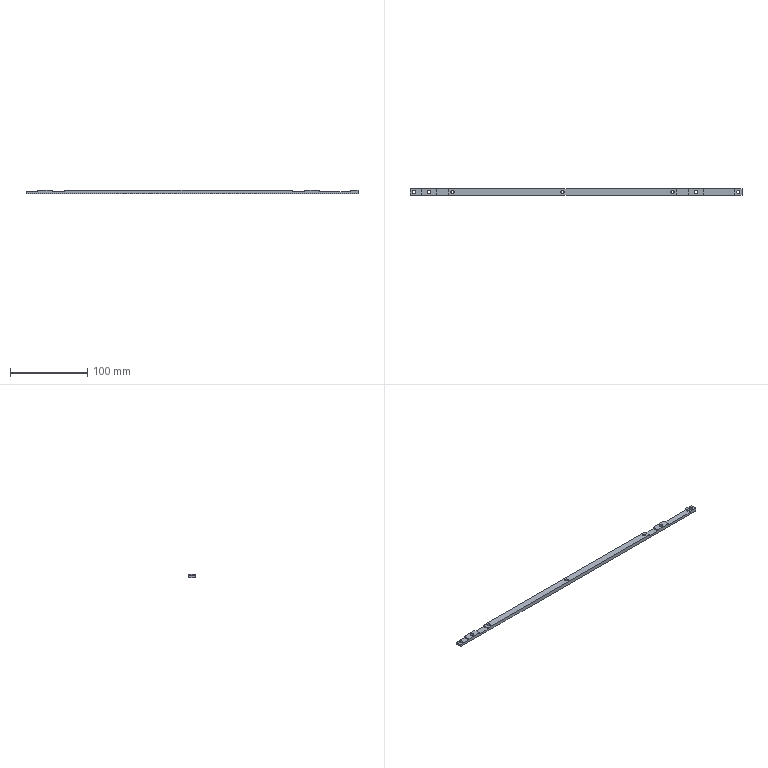CAM job | Mastercam | mm | 5 operations | part box 434.5 x 27.75 x 5
1. Facing | 9 - 10 平铣刀
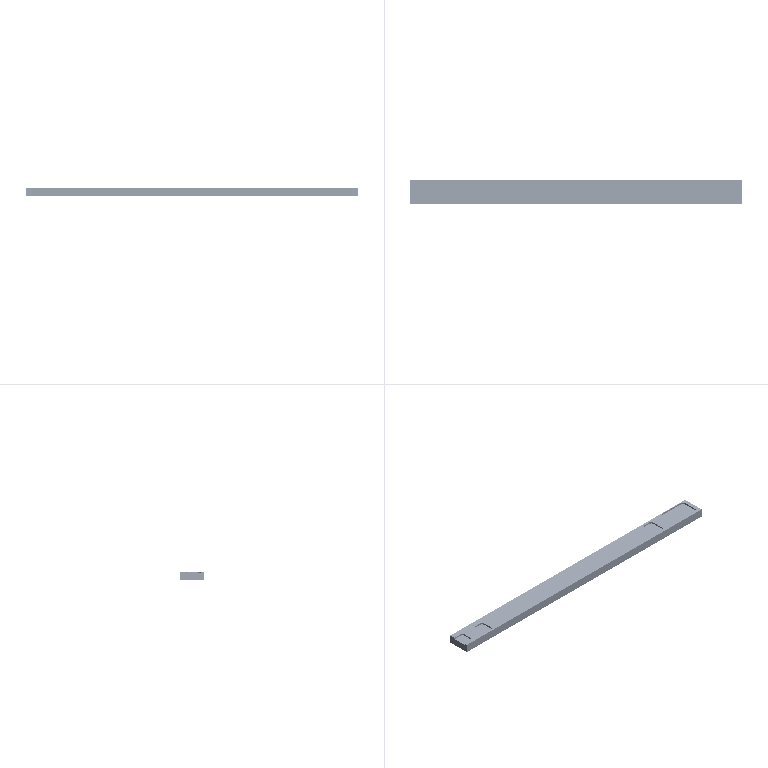2. Contour (2D) | 2 - 6 平铣刀
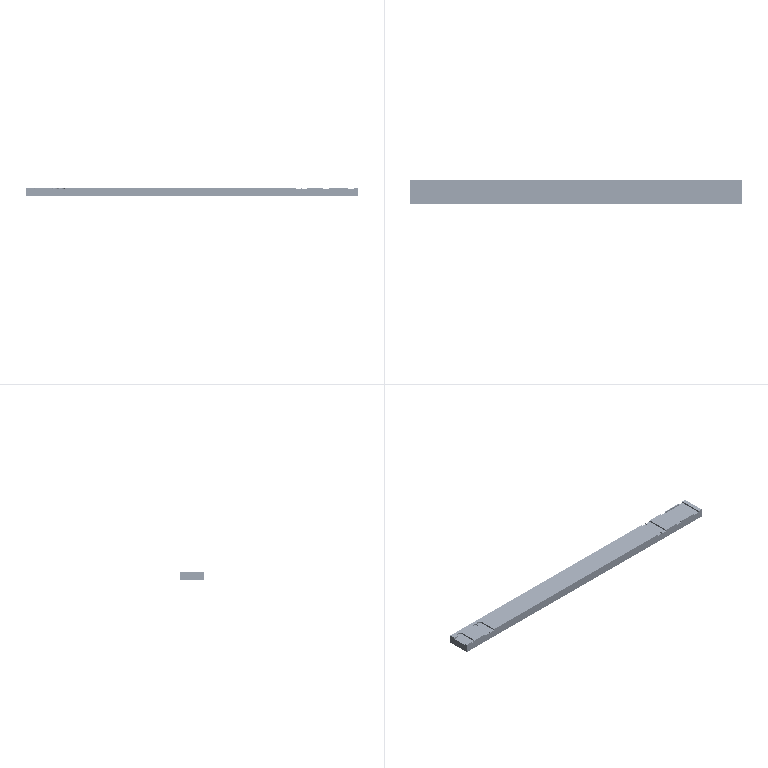3. Drill/Counterbore | 12 - 12 定位钻
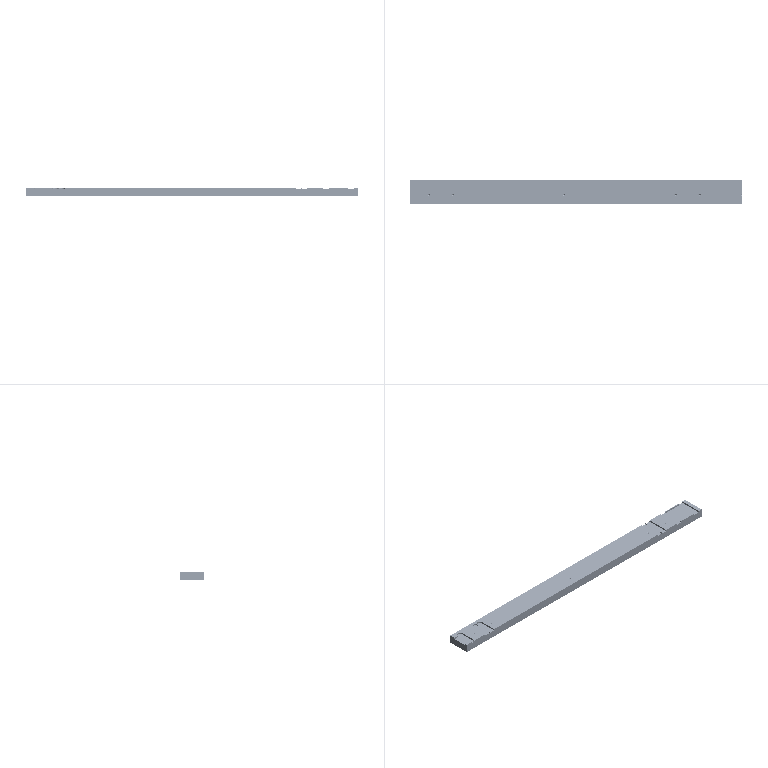4. Drill/Counterbore | 12 - 12 定位钻
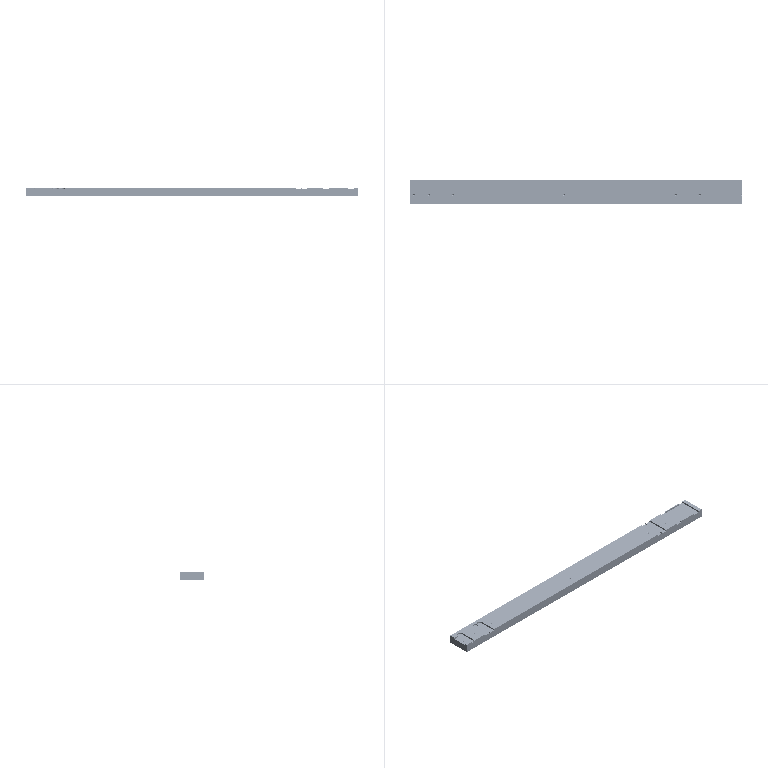5. Peck Drill | 11 - 4.3 钻头